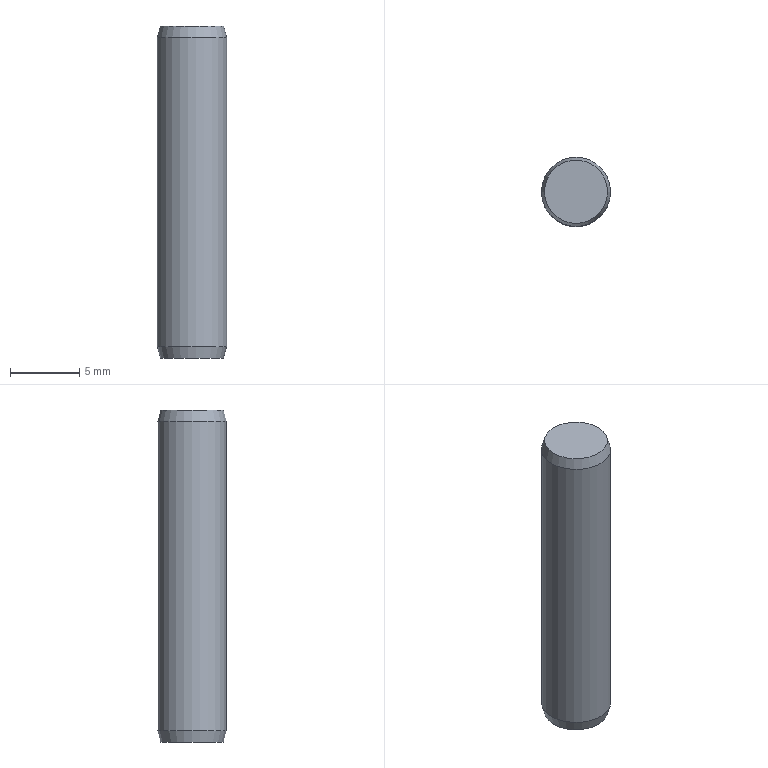Component | NX | GB-T119_1-2000_5X24_2 | 1 solid | 5 faces | box 5 x 5 x 24 mm | volume 469 mm3 | plane 2 | cone 2 | cylinder 1 | commonest cylinder face diameters 5 x1
STEP:
#1=CARTESIAN_POINT('',(0.,0.,0.));
#2=DIRECTION('',(0.,0.,1.));
#3=DIRECTION('',(1.,0.,0.));
#4=AXIS2_PLACEMENT_3D('',#1,#2,#3);
#5=CARTESIAN_POINT('',(-46.286,17.5,14.));
#6=VERTEX_POINT('',#5);
#7=CARTESIAN_POINT('',(-44.,17.5,14.));
#8=DIRECTION('',(0.,0.,-1.));
#9=DIRECTION('',(-1.,0.,0.));
#10=AXIS2_PLACEMENT_3D('',#7,#8,#9);
#11=CIRCLE('',#10,2.286);
#12=CARTESIAN_POINT('',(-44.,17.5,14.));
#13=DIRECTION('',(0.,0.,-1.));
#14=DIRECTION('',(-1.,0.,0.));
#15=AXIS2_PLACEMENT_3D('',#12,#13,#14);
#16=PLANE('',#15);
#17=CARTESIAN_POINT('',(0.,0.));
#18=DIRECTION('',(1.,0.));
#19=AXIS2_PLACEMENT_2D('',#17,#18);
#20=CIRCLE('',#19,2.286);
#21=(GEOMETRIC_REPRESENTATION_CONTEXT(2)PARAMETRIC_REPRESENTATION_CONTEXT()REPRESENTATION_CONTEXT('',''));
#22=DEFINITIONAL_REPRESENTATION('',(#20),#21);
#23=PCURVE('',#16,#22);
#24=CARTESIAN_POINT('',(-44.,17.5,14.));
#25=DIRECTION('',(0.,0.,1.));
#26=DIRECTION('',(1.,0.,0.));
#27=AXIS2_PLACEMENT_3D('',#24,#25,#26);
#28=CONICAL_SURFACE('',#27,2.286,0.2618);
#29=CARTESIAN_POINT('',(9.425,-0.));
#30=DIRECTION('',(-1.,0.));
#31=VECTOR('',#30,1.);
#32=LINE('',#29,#31);
#33=(GEOMETRIC_REPRESENTATION_CONTEXT(2)PARAMETRIC_REPRESENTATION_CONTEXT()REPRESENTATION_CONTEXT('',''));
#34=DEFINITIONAL_REPRESENTATION('',(#32),#33);
#35=PCURVE('',#28,#34);
#36=SURFACE_CURVE('',#11,(#23,#35),.PCURVE_S1.);
#37=EDGE_CURVE('',#6,#6,#36,.T.);
#38=ORIENTED_EDGE('',*,*,#37,.T.);
#39=EDGE_LOOP('',(#38));
#40=FACE_BOUND('',#39,.T.);
#41=ADVANCED_FACE('',(#40),#16,.T.);
#42=CARTESIAN_POINT('',(-46.5,17.5,14.8));
#43=VERTEX_POINT('',#42);
#44=CARTESIAN_POINT('',(-44.,17.5,14.8));
#45=DIRECTION('',(0.,0.,-1.));
#46=DIRECTION('',(-1.,0.,0.));
#47=AXIS2_PLACEMENT_3D('',#44,#45,#46);
#48=CIRCLE('',#47,2.5);
#49=CARTESIAN_POINT('',(9.425,0.8));
#50=DIRECTION('',(-1.,0.));
#51=VECTOR('',#50,1.);
#52=LINE('',#49,#51);
#53=(GEOMETRIC_REPRESENTATION_CONTEXT(2)PARAMETRIC_REPRESENTATION_CONTEXT()REPRESENTATION_CONTEXT('',''));
#54=DEFINITIONAL_REPRESENTATION('',(#52),#53);
#55=PCURVE('',#28,#54);
#56=CARTESIAN_POINT('',(-44.,17.5,38.));
#57=DIRECTION('',(0.,0.,-1.));
#58=DIRECTION('',(-1.,0.,0.));
#59=AXIS2_PLACEMENT_3D('',#56,#57,#58);
#60=CYLINDRICAL_SURFACE('',#59,2.5);
#61=CARTESIAN_POINT('',(0.,23.2));
#62=DIRECTION('',(1.,0.));
#63=VECTOR('',#62,1.);
#64=LINE('',#61,#63);
#65=(GEOMETRIC_REPRESENTATION_CONTEXT(2)PARAMETRIC_REPRESENTATION_CONTEXT()REPRESENTATION_CONTEXT('',''));
#66=DEFINITIONAL_REPRESENTATION('',(#64),#65);
#67=PCURVE('',#60,#66);
#68=SURFACE_CURVE('',#48,(#55,#67),.PCURVE_S1.);
#69=EDGE_CURVE('',#43,#43,#68,.T.);
#70=ORIENTED_EDGE('',*,*,#69,.T.);
#71=CARTESIAN_POINT('',(-46.286,17.5,14.));
#72=CARTESIAN_POINT('',(-46.5,17.5,14.8));
#73=B_SPLINE_CURVE_WITH_KNOTS('',1,(#71,#72),.UNSPECIFIED.,.F.,.F.,(2,2),(-0.,0.8282),.PIECEWISE_BEZIER_KNOTS.);
#74=CARTESIAN_POINT('',(3.142,0.));
#75=DIRECTION('',(0.,1.));
#76=VECTOR('',#75,1.);
#77=LINE('',#74,#76);
#78=(GEOMETRIC_REPRESENTATION_CONTEXT(2)PARAMETRIC_REPRESENTATION_CONTEXT()REPRESENTATION_CONTEXT('',''));
#79=DEFINITIONAL_REPRESENTATION('',(#77),#78);
#80=PCURVE('',#28,#79);
#81=CARTESIAN_POINT('',(9.425,0.));
#82=DIRECTION('',(0.,1.));
#83=VECTOR('',#82,1.);
#84=LINE('',#81,#83);
#85=(GEOMETRIC_REPRESENTATION_CONTEXT(2)PARAMETRIC_REPRESENTATION_CONTEXT()REPRESENTATION_CONTEXT('',''));
#86=DEFINITIONAL_REPRESENTATION('',(#84),#85);
#87=PCURVE('',#28,#86);
#88=SEAM_CURVE('',#73,(#80,#87),.PCURVE_S1.);
#89=EDGE_CURVE('',#6,#43,#88,.T.);
#90=ORIENTED_EDGE('',*,*,#89,.F.);
#91=ORIENTED_EDGE('',*,*,#37,.F.);
#92=ORIENTED_EDGE('',*,*,#89,.T.);
#93=EDGE_LOOP('',(#70,#90,#91,#92));
#94=FACE_BOUND('',#93,.T.);
#95=ADVANCED_FACE('',(#94),#28,.T.);
#96=CARTESIAN_POINT('',(-46.5,17.5,37.2));
#97=VERTEX_POINT('',#96);
#98=CARTESIAN_POINT('',(-44.,17.5,37.2));
#99=DIRECTION('',(0.,0.,-1.));
#100=DIRECTION('',(-1.,0.,0.));
#101=AXIS2_PLACEMENT_3D('',#98,#99,#100);
#102=CIRCLE('',#101,2.5);
#103=CARTESIAN_POINT('',(0.,0.8));
#104=DIRECTION('',(1.,0.));
#105=VECTOR('',#104,1.);
#106=LINE('',#103,#105);
#107=(GEOMETRIC_REPRESENTATION_CONTEXT(2)PARAMETRIC_REPRESENTATION_CONTEXT()REPRESENTATION_CONTEXT('',''));
#108=DEFINITIONAL_REPRESENTATION('',(#106),#107);
#109=PCURVE('',#60,#108);
#110=CARTESIAN_POINT('',(-44.,17.5,37.2));
#111=DIRECTION('',(0.,0.,-1.));
#112=DIRECTION('',(-1.,0.,0.));
#113=AXIS2_PLACEMENT_3D('',#110,#111,#112);
#114=CONICAL_SURFACE('',#113,2.5,0.2618);
#115=CARTESIAN_POINT('',(0.,-0.));
#116=DIRECTION('',(1.,0.));
#117=VECTOR('',#116,1.);
#118=LINE('',#115,#117);
#119=(GEOMETRIC_REPRESENTATION_CONTEXT(2)PARAMETRIC_REPRESENTATION_CONTEXT()REPRESENTATION_CONTEXT('',''));
#120=DEFINITIONAL_REPRESENTATION('',(#118),#119);
#121=PCURVE('',#114,#120);
#122=SURFACE_CURVE('',#102,(#109,#121),.PCURVE_S1.);
#123=EDGE_CURVE('',#97,#97,#122,.T.);
#124=ORIENTED_EDGE('',*,*,#123,.T.);
#125=CARTESIAN_POINT('',(-46.5,17.5,37.2));
#126=CARTESIAN_POINT('',(-46.5,17.5,14.8));
#127=B_SPLINE_CURVE_WITH_KNOTS('',1,(#125,#126),.UNSPECIFIED.,.F.,.F.,(2,2),(0.8,23.2),.PIECEWISE_BEZIER_KNOTS.);
#128=CARTESIAN_POINT('',(6.283,0.));
#129=DIRECTION('',(0.,1.));
#130=VECTOR('',#129,1.);
#131=LINE('',#128,#130);
#132=(GEOMETRIC_REPRESENTATION_CONTEXT(2)PARAMETRIC_REPRESENTATION_CONTEXT()REPRESENTATION_CONTEXT('',''));
#133=DEFINITIONAL_REPRESENTATION('',(#131),#132);
#134=PCURVE('',#60,#133);
#135=CARTESIAN_POINT('',(0.,0.));
#136=DIRECTION('',(0.,1.));
#137=VECTOR('',#136,1.);
#138=LINE('',#135,#137);
#139=(GEOMETRIC_REPRESENTATION_CONTEXT(2)PARAMETRIC_REPRESENTATION_CONTEXT()REPRESENTATION_CONTEXT('',''));
#140=DEFINITIONAL_REPRESENTATION('',(#138),#139);
#141=PCURVE('',#60,#140);
#142=SEAM_CURVE('',#127,(#134,#141),.PCURVE_S1.);
#143=EDGE_CURVE('',#97,#43,#142,.T.);
#144=ORIENTED_EDGE('',*,*,#143,.T.);
#145=ORIENTED_EDGE('',*,*,#69,.F.);
#146=ORIENTED_EDGE('',*,*,#143,.F.);
#147=EDGE_LOOP('',(#124,#144,#145,#146));
#148=FACE_BOUND('',#147,.T.);
#149=ADVANCED_FACE('',(#148),#60,.T.);
#150=CARTESIAN_POINT('',(-46.286,17.5,38.));
#151=VERTEX_POINT('',#150);
#152=CARTESIAN_POINT('',(-44.,17.5,38.));
#153=DIRECTION('',(0.,0.,-1.));
#154=DIRECTION('',(-1.,0.,0.));
#155=AXIS2_PLACEMENT_3D('',#152,#153,#154);
#156=CIRCLE('',#155,2.286);
#157=CARTESIAN_POINT('',(0.,-0.8));
#158=DIRECTION('',(1.,0.));
#159=VECTOR('',#158,1.);
#160=LINE('',#157,#159);
#161=(GEOMETRIC_REPRESENTATION_CONTEXT(2)PARAMETRIC_REPRESENTATION_CONTEXT()REPRESENTATION_CONTEXT('',''));
#162=DEFINITIONAL_REPRESENTATION('',(#160),#161);
#163=PCURVE('',#114,#162);
#164=CARTESIAN_POINT('',(-41.714,17.5,38.));
#165=DIRECTION('',(0.,0.,1.));
#166=DIRECTION('',(1.,0.,0.));
#167=AXIS2_PLACEMENT_3D('',#164,#165,#166);
#168=PLANE('',#167);
#169=CARTESIAN_POINT('',(-4.571,0.));
#170=CARTESIAN_POINT('',(-4.571,3.959));
#171=CARTESIAN_POINT('',(-1.143,1.979));
#172=CARTESIAN_POINT('',(2.286,0.));
#173=CARTESIAN_POINT('',(-1.143,-1.979));
#174=CARTESIAN_POINT('',(-4.571,-3.959));
#175=CARTESIAN_POINT('',(-4.571,0.));
#176=(BOUNDED_CURVE()B_SPLINE_CURVE(2,(#169,#170,#171,#172,#173,#174,#175),.UNSPECIFIED.,.T.,.F.)B_SPLINE_CURVE_WITH_KNOTS((1,2,2,2,2,1),(-2.094,0.,2.094,4.189,6.283,8.378),.UNSPECIFIED.)CURVE()GEOMETRIC_REPRESENTATION_ITEM()RATIONAL_B_SPLINE_CURVE((1.,0.5,1.,0.5,1.,0.5,1.))REPRESENTATION_ITEM(''));
#177=(GEOMETRIC_REPRESENTATION_CONTEXT(2)PARAMETRIC_REPRESENTATION_CONTEXT()REPRESENTATION_CONTEXT('',''));
#178=DEFINITIONAL_REPRESENTATION('',(#176),#177);
#179=PCURVE('',#168,#178);
#180=SURFACE_CURVE('',#156,(#163,#179),.PCURVE_S1.);
#181=EDGE_CURVE('',#151,#151,#180,.T.);
#182=ORIENTED_EDGE('',*,*,#181,.T.);
#183=CARTESIAN_POINT('',(-46.286,17.5,38.));
#184=CARTESIAN_POINT('',(-46.5,17.5,37.2));
#185=B_SPLINE_CURVE_WITH_KNOTS('',1,(#183,#184),.UNSPECIFIED.,.F.,.F.,(2,2),(-0.8282,-0.),.PIECEWISE_BEZIER_KNOTS.);
#186=CARTESIAN_POINT('',(6.283,0.));
#187=DIRECTION('',(0.,1.));
#188=VECTOR('',#187,1.);
#189=LINE('',#186,#188);
#190=(GEOMETRIC_REPRESENTATION_CONTEXT(2)PARAMETRIC_REPRESENTATION_CONTEXT()REPRESENTATION_CONTEXT('',''));
#191=DEFINITIONAL_REPRESENTATION('',(#189),#190);
#192=PCURVE('',#114,#191);
#193=CARTESIAN_POINT('',(0.,0.));
#194=DIRECTION('',(0.,1.));
#195=VECTOR('',#194,1.);
#196=LINE('',#193,#195);
#197=(GEOMETRIC_REPRESENTATION_CONTEXT(2)PARAMETRIC_REPRESENTATION_CONTEXT()REPRESENTATION_CONTEXT('',''));
#198=DEFINITIONAL_REPRESENTATION('',(#196),#197);
#199=PCURVE('',#114,#198);
#200=SEAM_CURVE('',#185,(#192,#199),.PCURVE_S1.);
#201=EDGE_CURVE('',#151,#97,#200,.T.);
#202=ORIENTED_EDGE('',*,*,#201,.T.);
#203=ORIENTED_EDGE('',*,*,#123,.F.);
#204=ORIENTED_EDGE('',*,*,#201,.F.);
#205=EDGE_LOOP('',(#182,#202,#203,#204));
#206=FACE_BOUND('',#205,.T.);
#207=ADVANCED_FACE('',(#206),#114,.T.);
#208=ORIENTED_EDGE('',*,*,#181,.F.);
#209=EDGE_LOOP('',(#208));
#210=FACE_BOUND('',#209,.T.);
#211=ADVANCED_FACE('',(#210),#168,.T.);
#212=CLOSED_SHELL('',(#41,#95,#149,#207,#211));
#213=MANIFOLD_SOLID_BREP('',#212);
#214=(LENGTH_UNIT()NAMED_UNIT(*)SI_UNIT(.MILLI.,.METRE.));
#215=UNCERTAINTY_MEASURE_WITH_UNIT(LENGTH_MEASURE(0.00001),#214,'','');
#216=(NAMED_UNIT(*)PLANE_ANGLE_UNIT()SI_UNIT($,.RADIAN.));
#217=(NAMED_UNIT(*)SI_UNIT($,.STERADIAN.)SOLID_ANGLE_UNIT());
#218=(GEOMETRIC_REPRESENTATION_CONTEXT(3)GLOBAL_UNCERTAINTY_ASSIGNED_CONTEXT((#215))GLOBAL_UNIT_ASSIGNED_CONTEXT((#214,#216,#217))REPRESENTATION_CONTEXT('',''));
#219=ADVANCED_BREP_SHAPE_REPRESENTATION('',(#4,#213),#218);